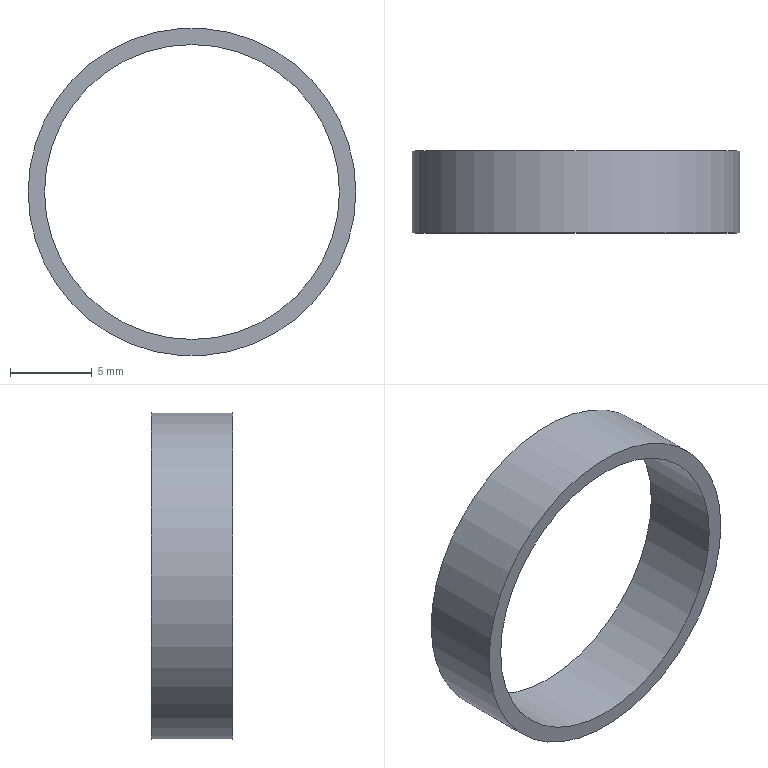Component | NX | BEARING | 1 solid | 4 faces | box 20 x 5 x 20 mm | volume 298 mm3 | cylinder 2 | plane 2 | commonest cylinder face diameters 20 x1 18 x1
STEP:
#1=CARTESIAN_POINT('',(0.,0.,0.));
#2=DIRECTION('',(0.,0.,1.));
#3=DIRECTION('',(1.,0.,0.));
#4=AXIS2_PLACEMENT_3D('',#1,#2,#3);
#5=CARTESIAN_POINT('',(-85.326,-192.61,50.));
#6=VERTEX_POINT('',#5);
#7=CARTESIAN_POINT('',(-95.326,-192.61,50.));
#8=DIRECTION('',(0.,-1.,0.));
#9=DIRECTION('',(1.,0.,0.));
#10=AXIS2_PLACEMENT_3D('',#7,#8,#9);
#11=CIRCLE('',#10,10.);
#12=CARTESIAN_POINT('',(-95.326,-192.61,50.));
#13=DIRECTION('',(0.,1.,0.));
#14=DIRECTION('',(-1.,0.,0.));
#15=AXIS2_PLACEMENT_3D('',#12,#13,#14);
#16=CYLINDRICAL_SURFACE('',#15,10.);
#17=CARTESIAN_POINT('',(9.425,0.));
#18=DIRECTION('',(-1.,0.));
#19=VECTOR('',#18,1.);
#20=LINE('',#17,#19);
#21=(GEOMETRIC_REPRESENTATION_CONTEXT(2)PARAMETRIC_REPRESENTATION_CONTEXT()REPRESENTATION_CONTEXT('',''));
#22=DEFINITIONAL_REPRESENTATION('',(#20),#21);
#23=PCURVE('',#16,#22);
#24=CARTESIAN_POINT('',(-95.326,-192.61,50.));
#25=DIRECTION('',(0.,-1.,0.));
#26=DIRECTION('',(1.,0.,0.));
#27=AXIS2_PLACEMENT_3D('',#24,#25,#26);
#28=PLANE('',#27);
#29=CARTESIAN_POINT('',(0.,0.));
#30=DIRECTION('',(1.,0.));
#31=AXIS2_PLACEMENT_2D('',#29,#30);
#32=CIRCLE('',#31,10.);
#33=(GEOMETRIC_REPRESENTATION_CONTEXT(2)PARAMETRIC_REPRESENTATION_CONTEXT()REPRESENTATION_CONTEXT('',''));
#34=DEFINITIONAL_REPRESENTATION('',(#32),#33);
#35=PCURVE('',#28,#34);
#36=SURFACE_CURVE('',#11,(#23,#35),.PCURVE_S1.);
#37=EDGE_CURVE('',#6,#6,#36,.T.);
#38=ORIENTED_EDGE('',*,*,#37,.F.);
#39=CARTESIAN_POINT('',(-85.326,-187.61,50.));
#40=VERTEX_POINT('',#39);
#41=CARTESIAN_POINT('',(-85.326,-192.61,50.));
#42=CARTESIAN_POINT('',(-85.326,-187.61,50.));
#43=B_SPLINE_CURVE_WITH_KNOTS('',1,(#41,#42),.UNSPECIFIED.,.F.,.F.,(2,2),(0.,5.),.PIECEWISE_BEZIER_KNOTS.);
#44=CARTESIAN_POINT('',(9.425,0.));
#45=DIRECTION('',(0.,1.));
#46=VECTOR('',#45,1.);
#47=LINE('',#44,#46);
#48=(GEOMETRIC_REPRESENTATION_CONTEXT(2)PARAMETRIC_REPRESENTATION_CONTEXT()REPRESENTATION_CONTEXT('',''));
#49=DEFINITIONAL_REPRESENTATION('',(#47),#48);
#50=PCURVE('',#16,#49);
#51=CARTESIAN_POINT('',(3.142,0.));
#52=DIRECTION('',(0.,1.));
#53=VECTOR('',#52,1.);
#54=LINE('',#51,#53);
#55=(GEOMETRIC_REPRESENTATION_CONTEXT(2)PARAMETRIC_REPRESENTATION_CONTEXT()REPRESENTATION_CONTEXT('',''));
#56=DEFINITIONAL_REPRESENTATION('',(#54),#55);
#57=PCURVE('',#16,#56);
#58=SEAM_CURVE('',#43,(#50,#57),.PCURVE_S1.);
#59=EDGE_CURVE('',#6,#40,#58,.T.);
#60=ORIENTED_EDGE('',*,*,#59,.T.);
#61=CARTESIAN_POINT('',(-95.326,-187.61,50.));
#62=DIRECTION('',(0.,-1.,0.));
#63=DIRECTION('',(1.,0.,0.));
#64=AXIS2_PLACEMENT_3D('',#61,#62,#63);
#65=CIRCLE('',#64,10.);
#66=CARTESIAN_POINT('',(9.425,5.));
#67=DIRECTION('',(-1.,0.));
#68=VECTOR('',#67,1.);
#69=LINE('',#66,#68);
#70=(GEOMETRIC_REPRESENTATION_CONTEXT(2)PARAMETRIC_REPRESENTATION_CONTEXT()REPRESENTATION_CONTEXT('',''));
#71=DEFINITIONAL_REPRESENTATION('',(#69),#70);
#72=PCURVE('',#16,#71);
#73=CARTESIAN_POINT('',(-95.326,-187.61,50.));
#74=DIRECTION('',(0.,-1.,0.));
#75=DIRECTION('',(1.,0.,0.));
#76=AXIS2_PLACEMENT_3D('',#73,#74,#75);
#77=PLANE('',#76);
#78=CARTESIAN_POINT('',(0.,0.));
#79=DIRECTION('',(1.,0.));
#80=AXIS2_PLACEMENT_2D('',#78,#79);
#81=CIRCLE('',#80,10.);
#82=(GEOMETRIC_REPRESENTATION_CONTEXT(2)PARAMETRIC_REPRESENTATION_CONTEXT()REPRESENTATION_CONTEXT('',''));
#83=DEFINITIONAL_REPRESENTATION('',(#81),#82);
#84=PCURVE('',#77,#83);
#85=SURFACE_CURVE('',#65,(#72,#84),.PCURVE_S1.);
#86=EDGE_CURVE('',#40,#40,#85,.T.);
#87=ORIENTED_EDGE('',*,*,#86,.T.);
#88=ORIENTED_EDGE('',*,*,#59,.F.);
#89=EDGE_LOOP('',(#38,#60,#87,#88));
#90=FACE_BOUND('',#89,.T.);
#91=ADVANCED_FACE('',(#90),#16,.T.);
#92=CARTESIAN_POINT('',(-86.326,-192.61,50.));
#93=VERTEX_POINT('',#92);
#94=CARTESIAN_POINT('',(-95.326,-192.61,50.));
#95=DIRECTION('',(0.,-1.,0.));
#96=DIRECTION('',(1.,0.,0.));
#97=AXIS2_PLACEMENT_3D('',#94,#95,#96);
#98=CIRCLE('',#97,9.);
#99=CARTESIAN_POINT('',(-95.326,-192.61,50.));
#100=DIRECTION('',(0.,1.,0.));
#101=DIRECTION('',(-1.,0.,0.));
#102=AXIS2_PLACEMENT_3D('',#99,#100,#101);
#103=CYLINDRICAL_SURFACE('',#102,9.);
#104=CARTESIAN_POINT('',(9.425,0.));
#105=DIRECTION('',(-1.,0.));
#106=VECTOR('',#105,1.);
#107=LINE('',#104,#106);
#108=(GEOMETRIC_REPRESENTATION_CONTEXT(2)PARAMETRIC_REPRESENTATION_CONTEXT()REPRESENTATION_CONTEXT('',''));
#109=DEFINITIONAL_REPRESENTATION('',(#107),#108);
#110=PCURVE('',#103,#109);
#111=CARTESIAN_POINT('',(0.,0.));
#112=DIRECTION('',(1.,0.));
#113=AXIS2_PLACEMENT_2D('',#111,#112);
#114=CIRCLE('',#113,9.);
#115=(GEOMETRIC_REPRESENTATION_CONTEXT(2)PARAMETRIC_REPRESENTATION_CONTEXT()REPRESENTATION_CONTEXT('',''));
#116=DEFINITIONAL_REPRESENTATION('',(#114),#115);
#117=PCURVE('',#28,#116);
#118=SURFACE_CURVE('',#98,(#110,#117),.PCURVE_S1.);
#119=EDGE_CURVE('',#93,#93,#118,.T.);
#120=ORIENTED_EDGE('',*,*,#119,.F.);
#121=CARTESIAN_POINT('',(-86.326,-187.61,50.));
#122=VERTEX_POINT('',#121);
#123=CARTESIAN_POINT('',(-86.326,-192.61,50.));
#124=CARTESIAN_POINT('',(-86.326,-187.61,50.));
#125=B_SPLINE_CURVE_WITH_KNOTS('',1,(#123,#124),.UNSPECIFIED.,.F.,.F.,(2,2),(0.,5.),.PIECEWISE_BEZIER_KNOTS.);
#126=CARTESIAN_POINT('',(9.425,0.));
#127=DIRECTION('',(0.,1.));
#128=VECTOR('',#127,1.);
#129=LINE('',#126,#128);
#130=(GEOMETRIC_REPRESENTATION_CONTEXT(2)PARAMETRIC_REPRESENTATION_CONTEXT()REPRESENTATION_CONTEXT('',''));
#131=DEFINITIONAL_REPRESENTATION('',(#129),#130);
#132=PCURVE('',#103,#131);
#133=CARTESIAN_POINT('',(3.142,0.));
#134=DIRECTION('',(0.,1.));
#135=VECTOR('',#134,1.);
#136=LINE('',#133,#135);
#137=(GEOMETRIC_REPRESENTATION_CONTEXT(2)PARAMETRIC_REPRESENTATION_CONTEXT()REPRESENTATION_CONTEXT('',''));
#138=DEFINITIONAL_REPRESENTATION('',(#136),#137);
#139=PCURVE('',#103,#138);
#140=SEAM_CURVE('',#125,(#132,#139),.PCURVE_S1.);
#141=EDGE_CURVE('',#93,#122,#140,.T.);
#142=ORIENTED_EDGE('',*,*,#141,.T.);
#143=CARTESIAN_POINT('',(-95.326,-187.61,50.));
#144=DIRECTION('',(0.,-1.,0.));
#145=DIRECTION('',(1.,0.,0.));
#146=AXIS2_PLACEMENT_3D('',#143,#144,#145);
#147=CIRCLE('',#146,9.);
#148=CARTESIAN_POINT('',(9.425,5.));
#149=DIRECTION('',(-1.,0.));
#150=VECTOR('',#149,1.);
#151=LINE('',#148,#150);
#152=(GEOMETRIC_REPRESENTATION_CONTEXT(2)PARAMETRIC_REPRESENTATION_CONTEXT()REPRESENTATION_CONTEXT('',''));
#153=DEFINITIONAL_REPRESENTATION('',(#151),#152);
#154=PCURVE('',#103,#153);
#155=CARTESIAN_POINT('',(0.,0.));
#156=DIRECTION('',(1.,0.));
#157=AXIS2_PLACEMENT_2D('',#155,#156);
#158=CIRCLE('',#157,9.);
#159=(GEOMETRIC_REPRESENTATION_CONTEXT(2)PARAMETRIC_REPRESENTATION_CONTEXT()REPRESENTATION_CONTEXT('',''));
#160=DEFINITIONAL_REPRESENTATION('',(#158),#159);
#161=PCURVE('',#77,#160);
#162=SURFACE_CURVE('',#147,(#154,#161),.PCURVE_S1.);
#163=EDGE_CURVE('',#122,#122,#162,.T.);
#164=ORIENTED_EDGE('',*,*,#163,.T.);
#165=ORIENTED_EDGE('',*,*,#141,.F.);
#166=EDGE_LOOP('',(#120,#142,#164,#165));
#167=FACE_BOUND('',#166,.F.);
#168=ADVANCED_FACE('',(#167),#103,.F.);
#169=ORIENTED_EDGE('',*,*,#37,.T.);
#170=EDGE_LOOP('',(#169));
#171=FACE_BOUND('',#170,.T.);
#172=ORIENTED_EDGE('',*,*,#119,.F.);
#173=EDGE_LOOP('',(#172));
#174=FACE_BOUND('',#173,.T.);
#175=ADVANCED_FACE('',(#171,#174),#28,.T.);
#176=ORIENTED_EDGE('',*,*,#86,.F.);
#177=EDGE_LOOP('',(#176));
#178=FACE_BOUND('',#177,.T.);
#179=ORIENTED_EDGE('',*,*,#163,.T.);
#180=EDGE_LOOP('',(#179));
#181=FACE_BOUND('',#180,.T.);
#182=ADVANCED_FACE('',(#178,#181),#77,.F.);
#183=CLOSED_SHELL('',(#91,#168,#175,#182));
#184=MANIFOLD_SOLID_BREP('',#183);
#185=(LENGTH_UNIT()NAMED_UNIT(*)SI_UNIT(.MILLI.,.METRE.));
#186=UNCERTAINTY_MEASURE_WITH_UNIT(LENGTH_MEASURE(0.00001),#185,'','');
#187=(NAMED_UNIT(*)PLANE_ANGLE_UNIT()SI_UNIT($,.RADIAN.));
#188=(NAMED_UNIT(*)SI_UNIT($,.STERADIAN.)SOLID_ANGLE_UNIT());
#189=(GEOMETRIC_REPRESENTATION_CONTEXT(3)GLOBAL_UNCERTAINTY_ASSIGNED_CONTEXT((#186))GLOBAL_UNIT_ASSIGNED_CONTEXT((#185,#187,#188))REPRESENTATION_CONTEXT('',''));
#190=ADVANCED_BREP_SHAPE_REPRESENTATION('',(#4,#184),#189);